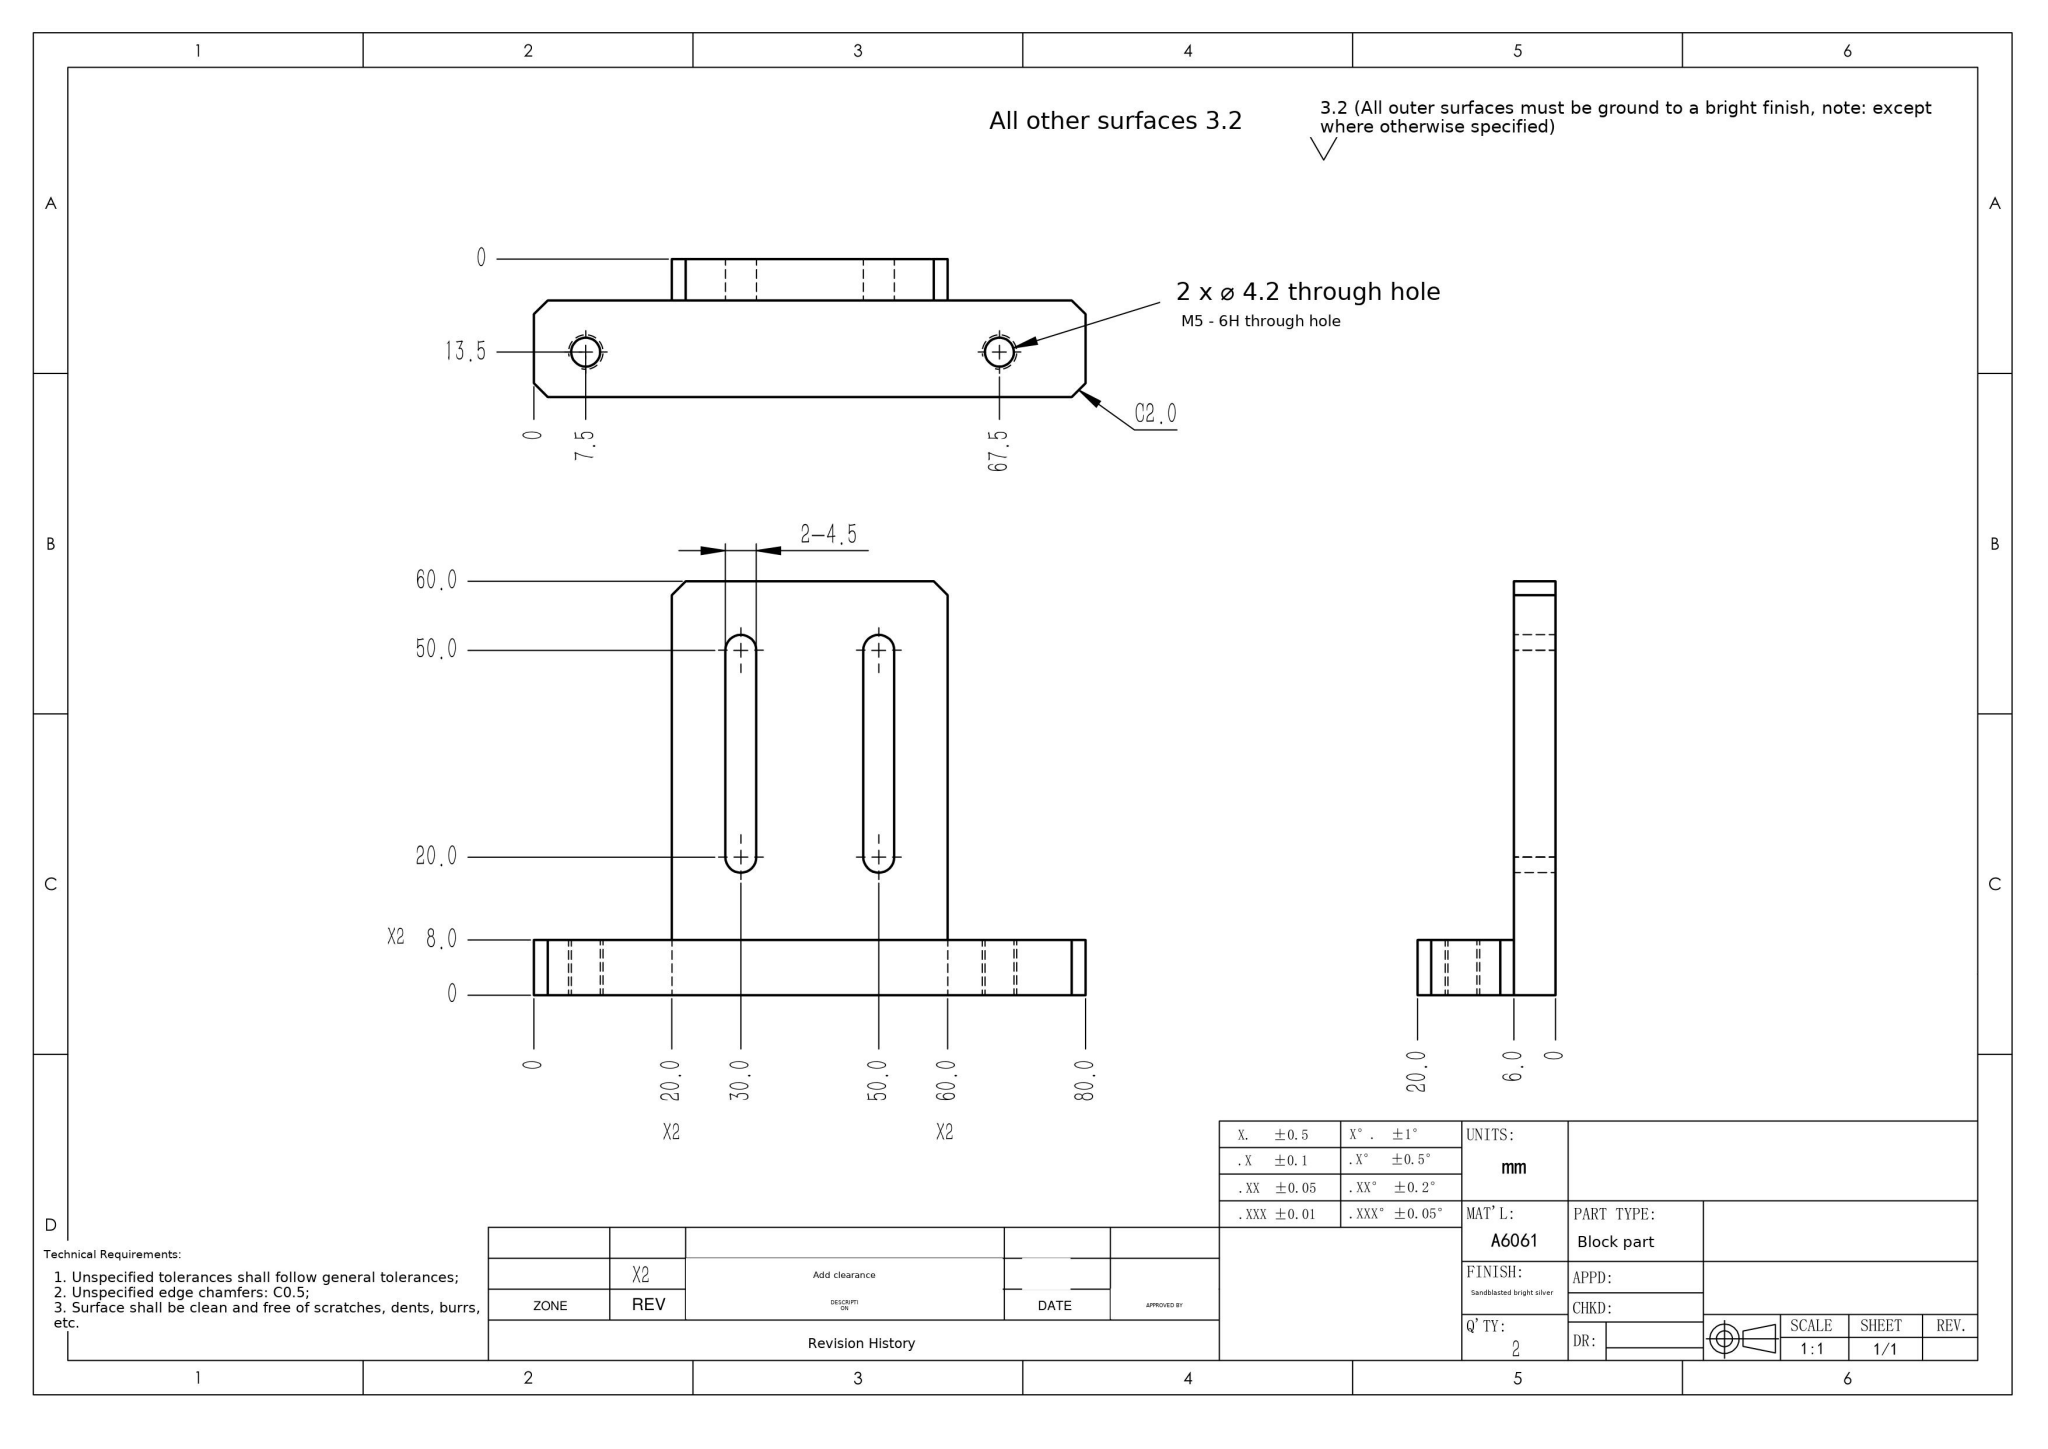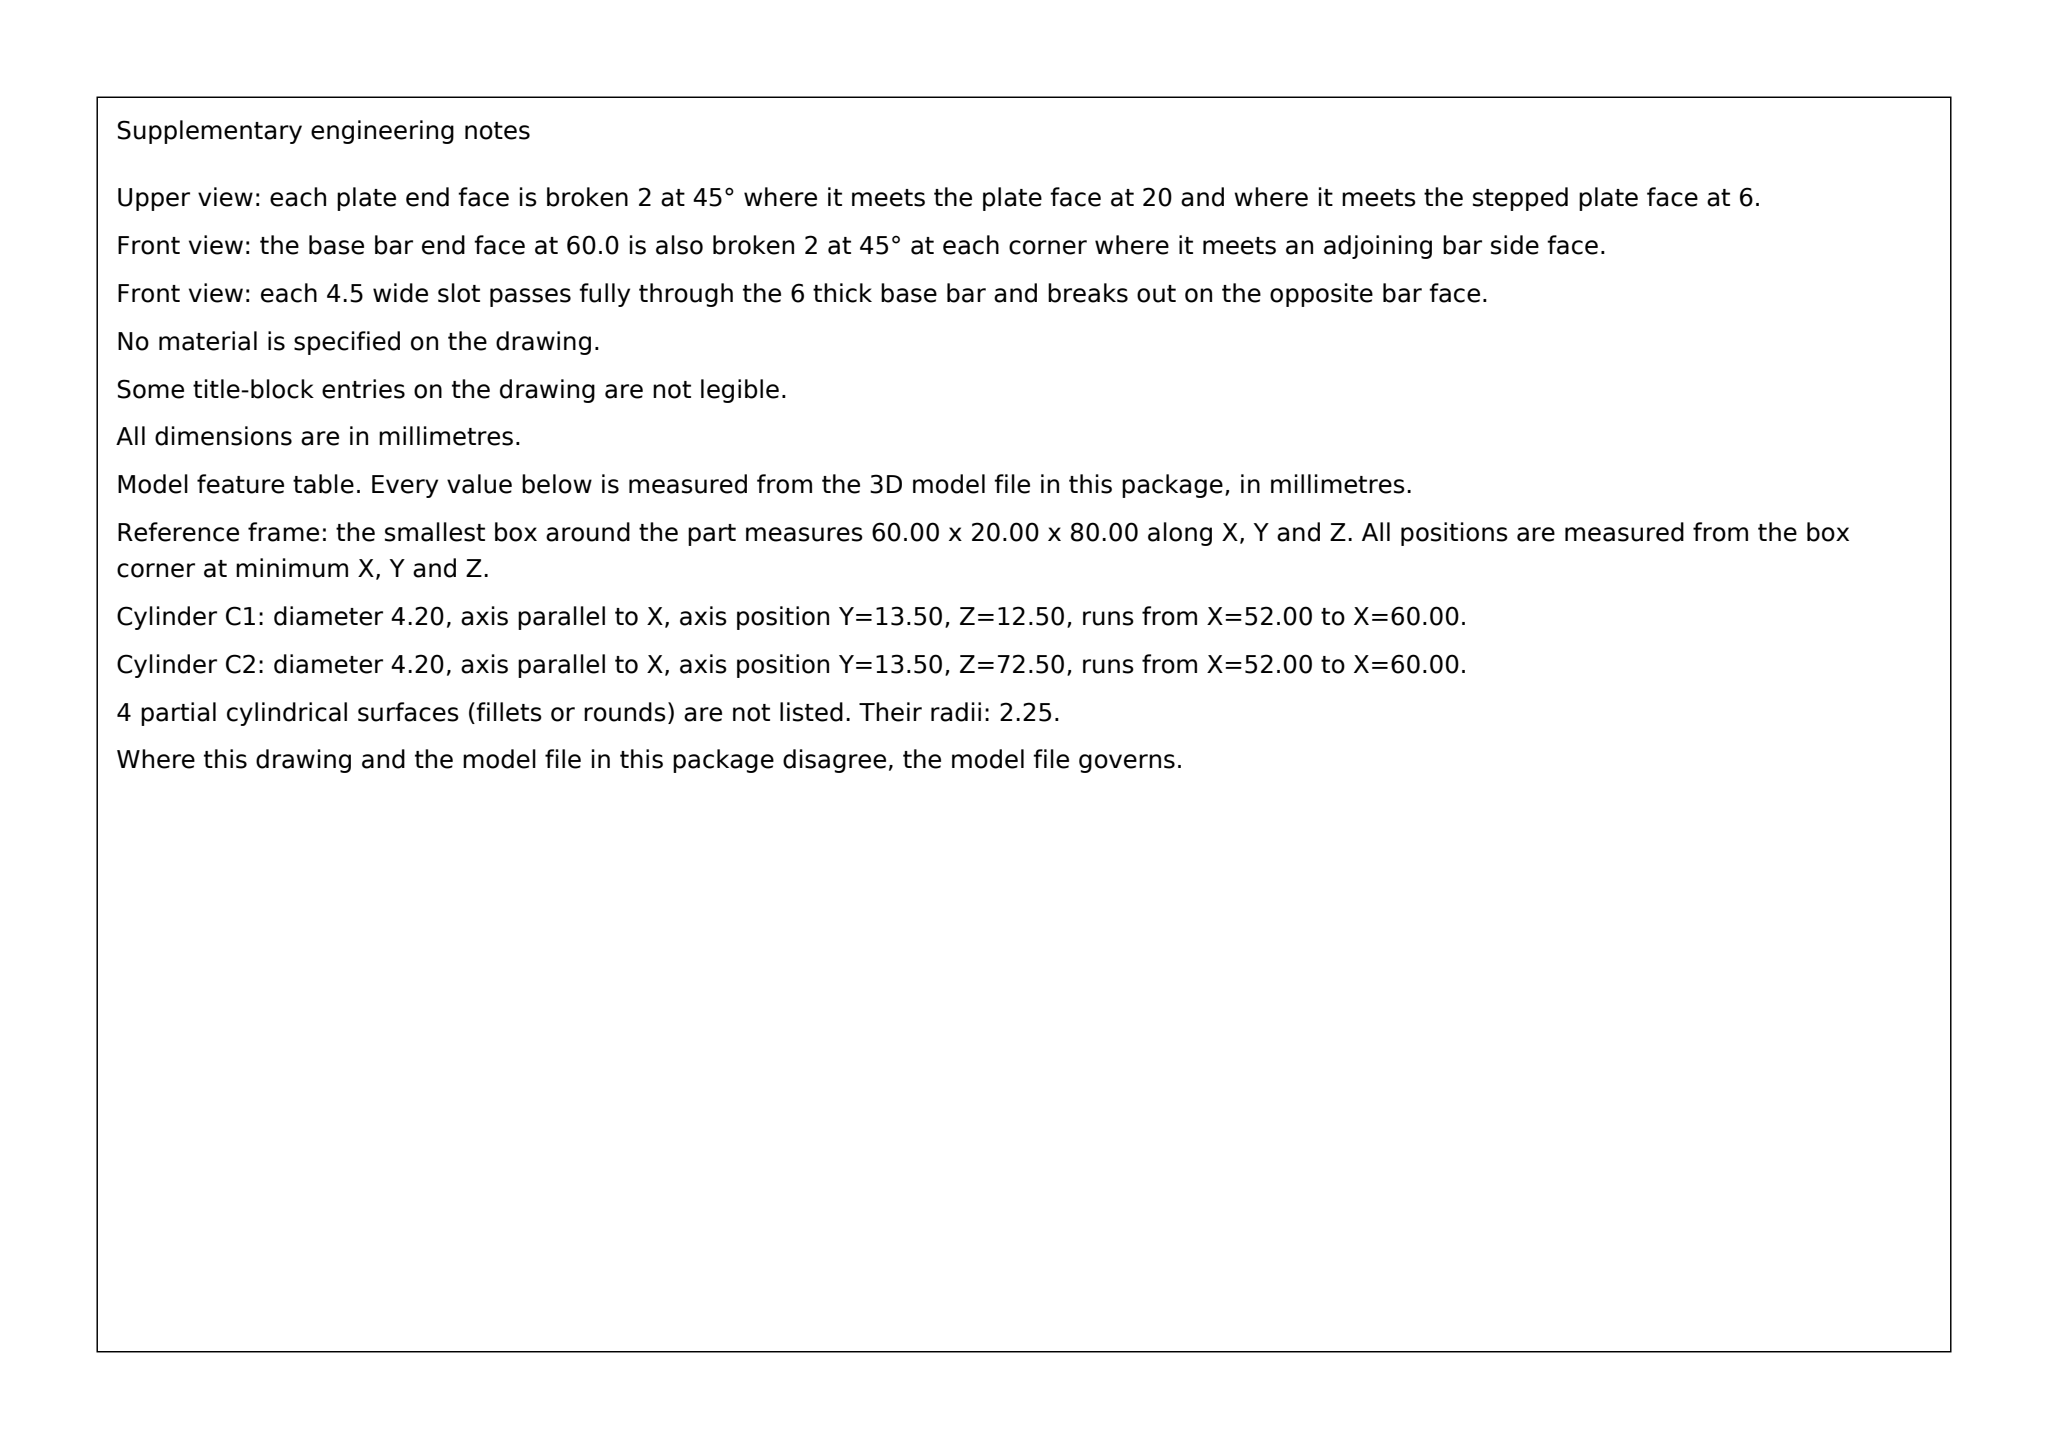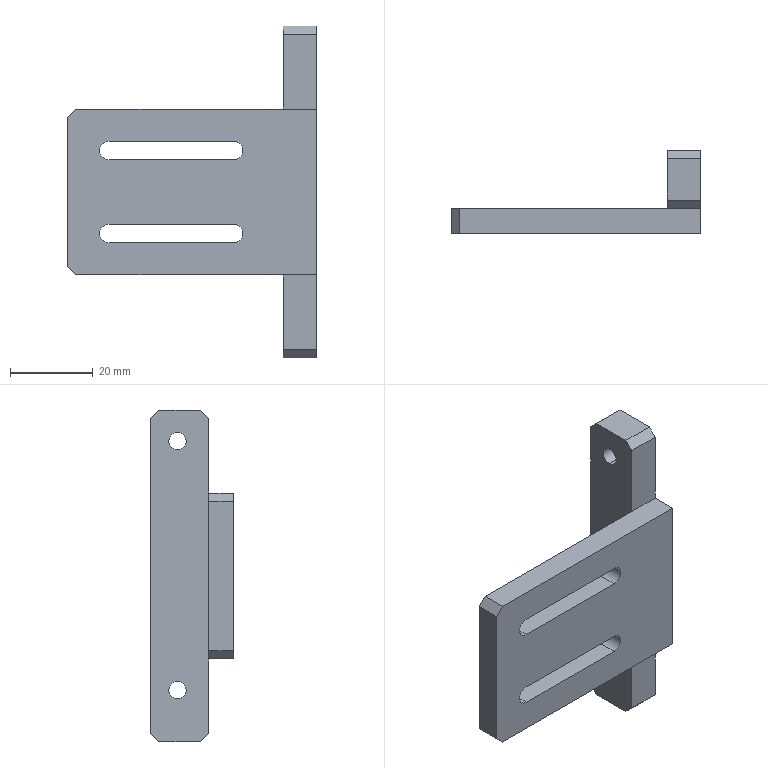Part | SolidWorks | mm | material A6061 | 1 solid | 32 faces | box 60 x 20 x 80 mm | volume 21239 mm3 | plane 22 | cylinder 10 | commonest cylinder face diameters 4.5 x6 4.2 x4
Drawing notes:
2X Ø4.2 THRU - CLEARANCE HOLE, NO THREAD (M5-6H NOT APPLIC) | from the solid: cylinders [4.2, axis x, (y=13.5, z=12.5) and (y=13.5, z=72.5), length 8.0] - plain straight bores, no thread/cone features in STEP
build123d program:
from build123d import *

# Parameters (mm, degrees)
BOSS_EXTRUDE1_DEPTH = 40
M5_TAPPED_HOLE1_D   = 4.2
CUT_EXTRUDE1_DEPTH  = 74.457
SKETCH7_W           = 20
SKETCH7_H           = 6
CUT_EXTRUDE2_DEPTH  = 75.833
CHAMFER1_SIZE       = 2


with BuildPart() as part:
    # Sketch1 → Boss-Extrude1 (new, symmetric)
    with BuildSketch(Plane.XY):
        Polygon((0, 0), (0, 20), (-8, 20), (-8, 6), (-60, 6), (-60, 0), align=None)
    extrude(amount=BOSS_EXTRUDE1_DEPTH, both=True)

    # M5 Tapped Hole1 (through all)
    with Locations(Plane(origin=(0, 0, 0), x_dir=(0, 0, -1), z_dir=(1, 0, 0))):
        with Locations((-32.5, 13.5), (27.5, 13.5)):
            Hole(M5_TAPPED_HOLE1_D / 2)

    # Sketch4 → Cut-Extrude1 (cut, through all)
    with BuildSketch(Plane(origin=(0, 6, 0), x_dir=(1, 0, 0), z_dir=(0, 1, 0))):
        with BuildLine():
            Line((-50, 12.25), (-20, 12.25))
            ThreePointArc((-20, 12.25), (-17.75, 10), (-20, 7.75))
            Line((-20, 7.75), (-50, 7.75))
            ThreePointArc((-50, 7.75), (-52.25, 10), (-50, 12.25))
        make_face()
        with BuildLine():
            Line((-50, -7.75), (-20, -7.75))
            ThreePointArc((-20, -7.75), (-17.75, -10), (-20, -12.25))
            Line((-20, -12.25), (-50, -12.25))
            ThreePointArc((-50, -12.25), (-52.25, -10), (-50, -7.75))
        make_face()
    extrude(amount=-CUT_EXTRUDE1_DEPTH, mode=Mode.SUBTRACT)

    # Sketch7 → Cut-Extrude2 (cut, through all)
    with BuildSketch(Plane(origin=(0, 0, 0), x_dir=(0, 0, -1), z_dir=(1, 0, 0))):
        with Locations((30, 3)):
            Rectangle(SKETCH7_W, SKETCH7_H)
        with Locations((-30, 3)):
            Rectangle(SKETCH7_W, SKETCH7_H)
    extrude(amount=-CUT_EXTRUDE2_DEPTH, mode=Mode.SUBTRACT)

    # Chamfer1
    chamfer1_edges = [part.edges().sort_by_distance(p)[0] for p in [
        (-4, 20, 40),
        (-4, 6, -40),
        (-60, 3, -20),
        (-4, 20, -40),
        (-4, 6, 40),
        (-60, 3, 20),
    ]]
    chamfer(chamfer1_edges, length=CHAMFER1_SIZE)


solid = part.part